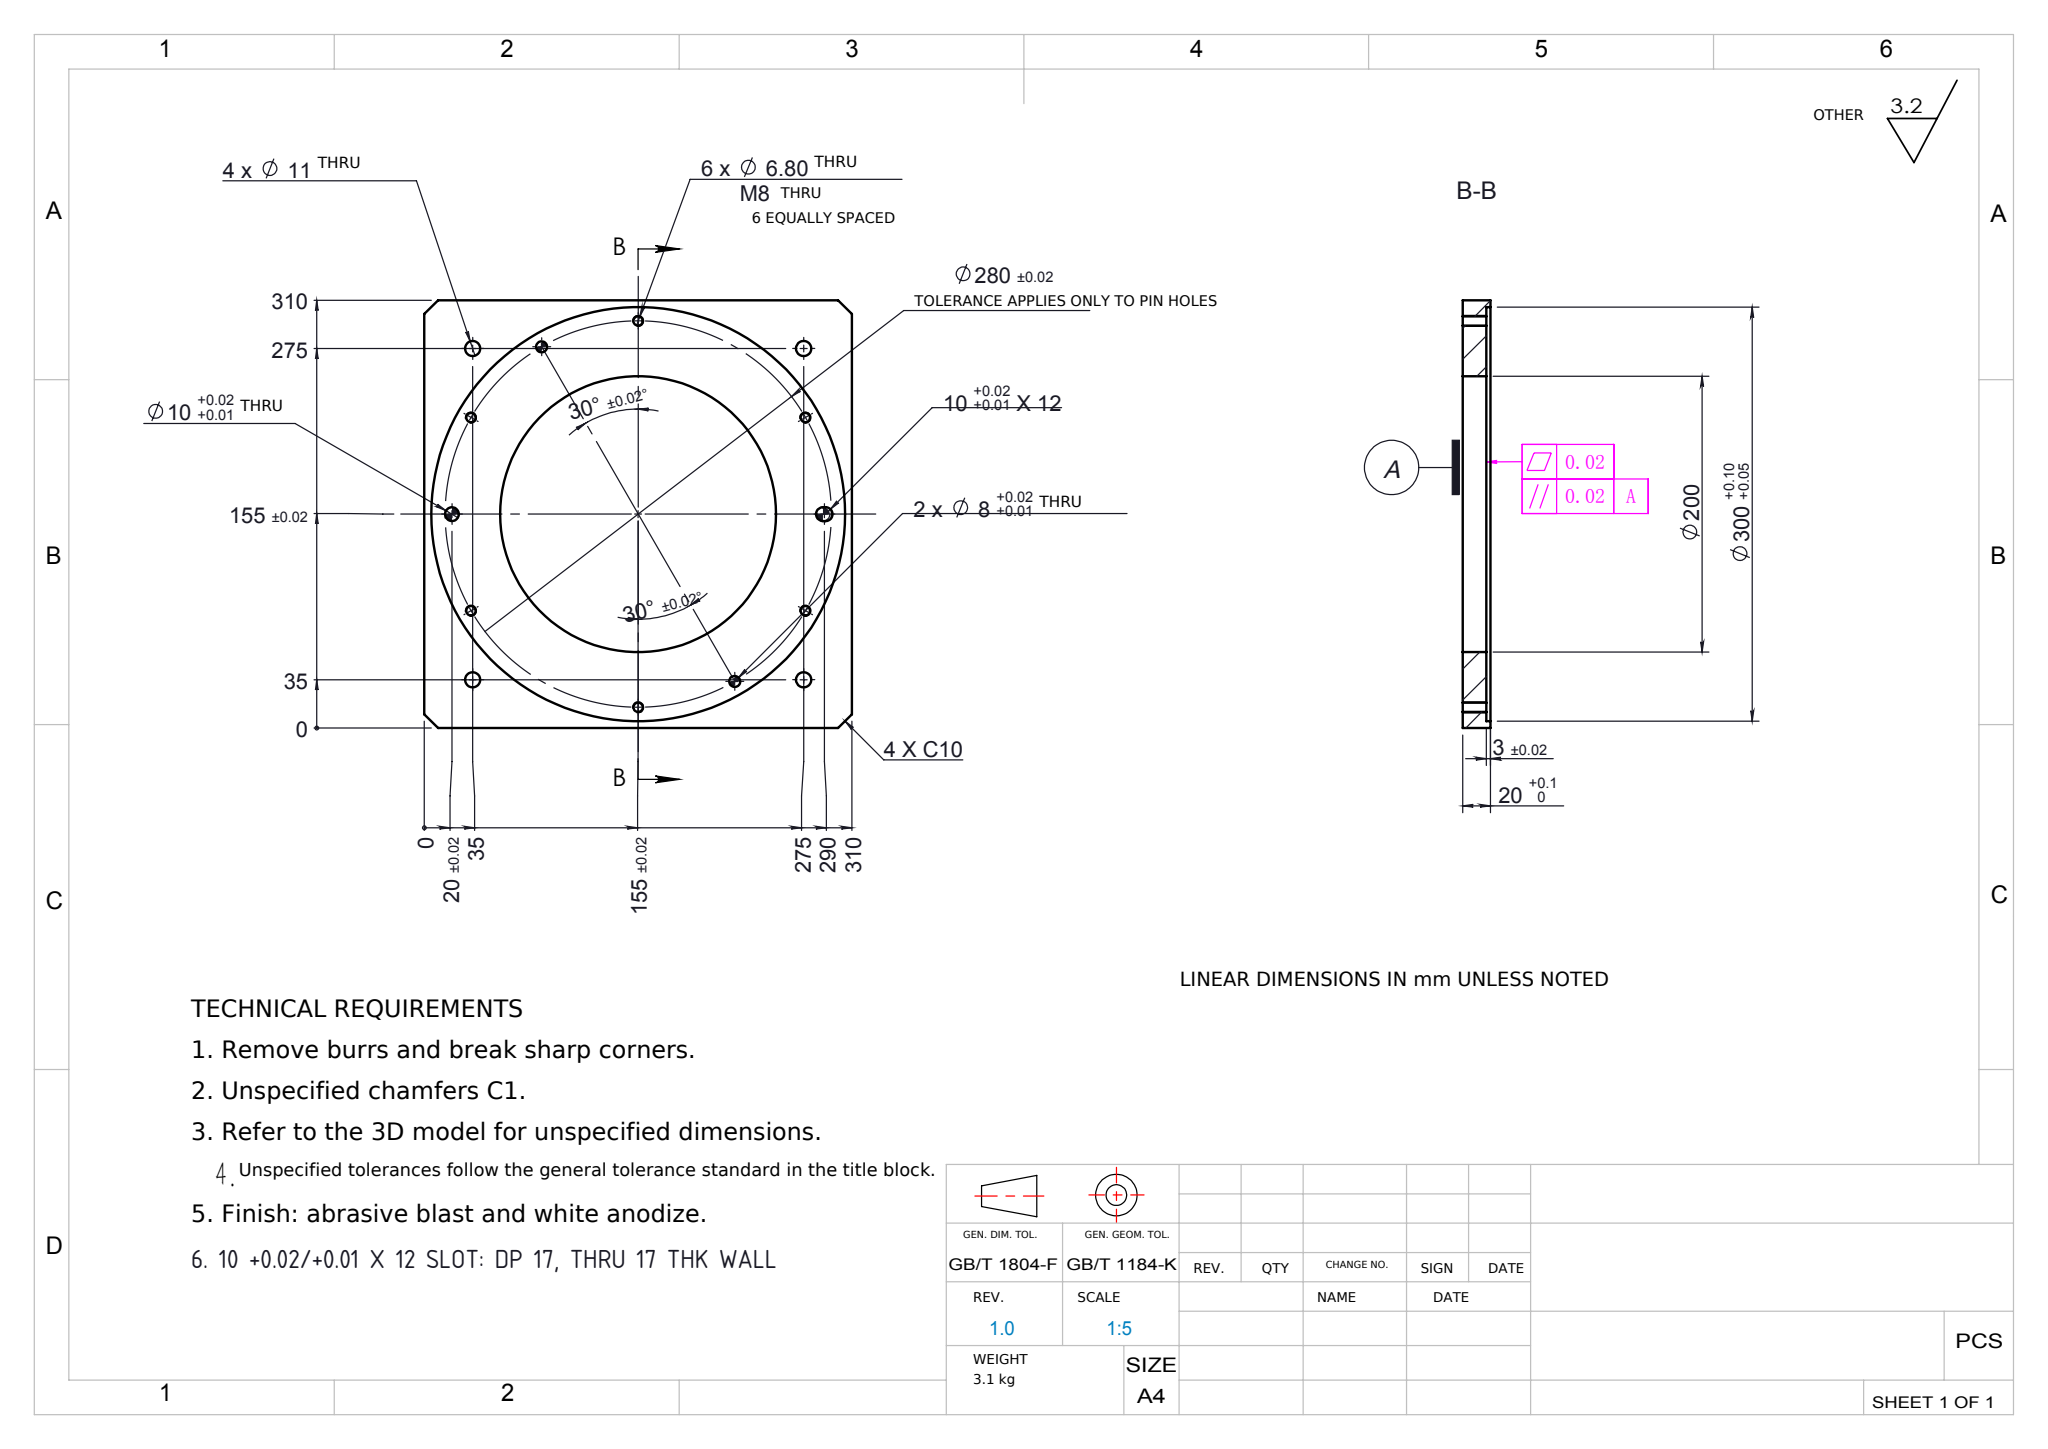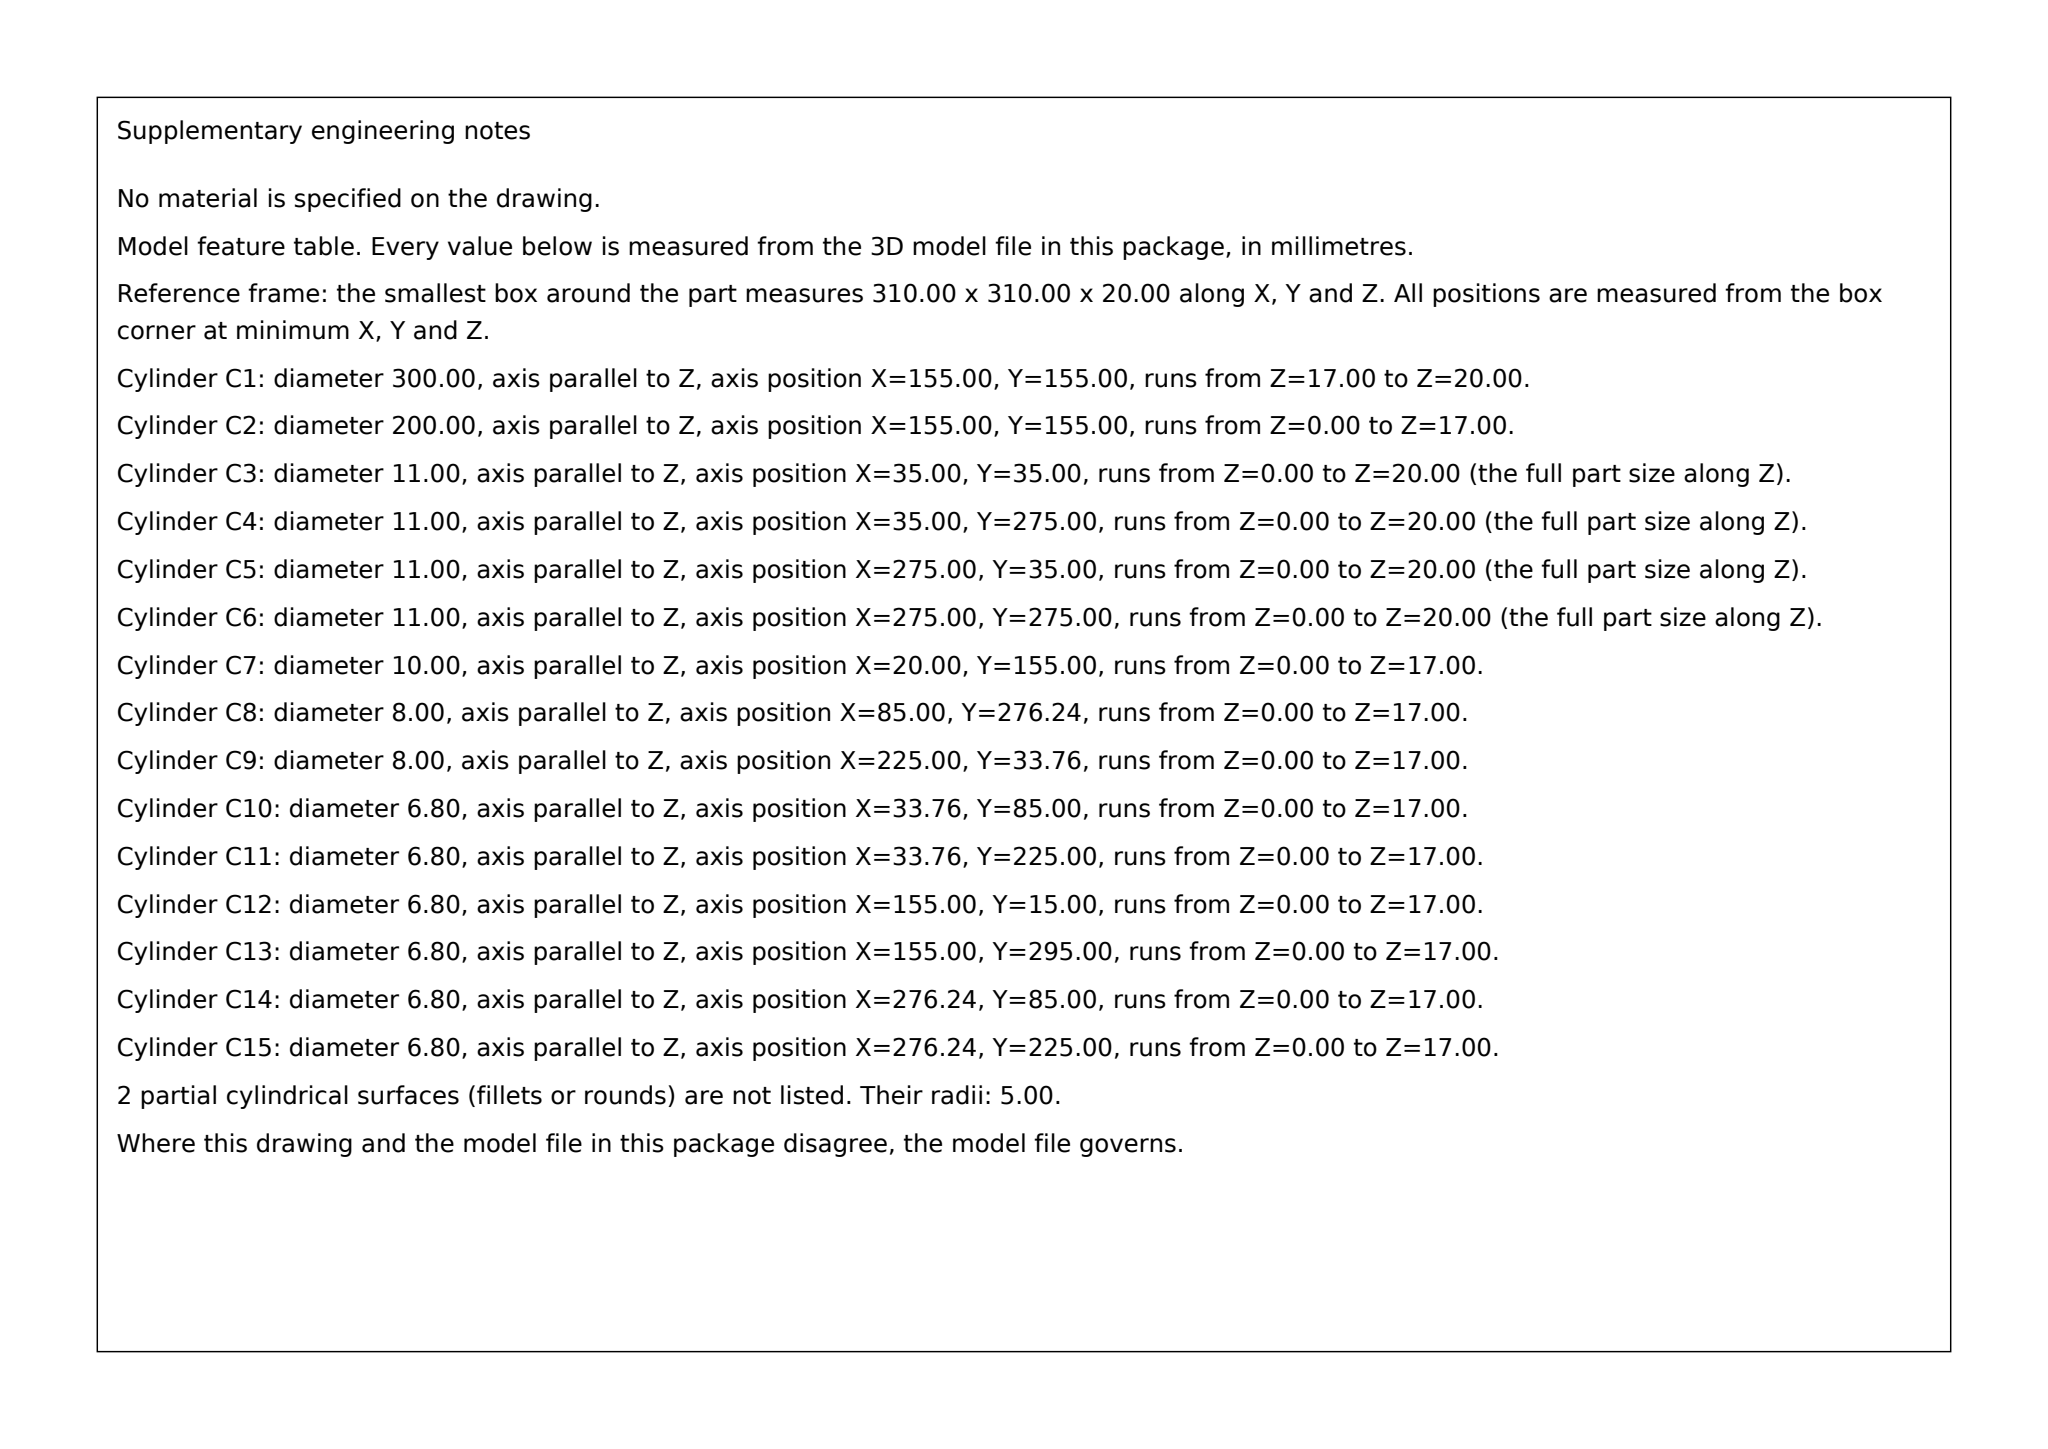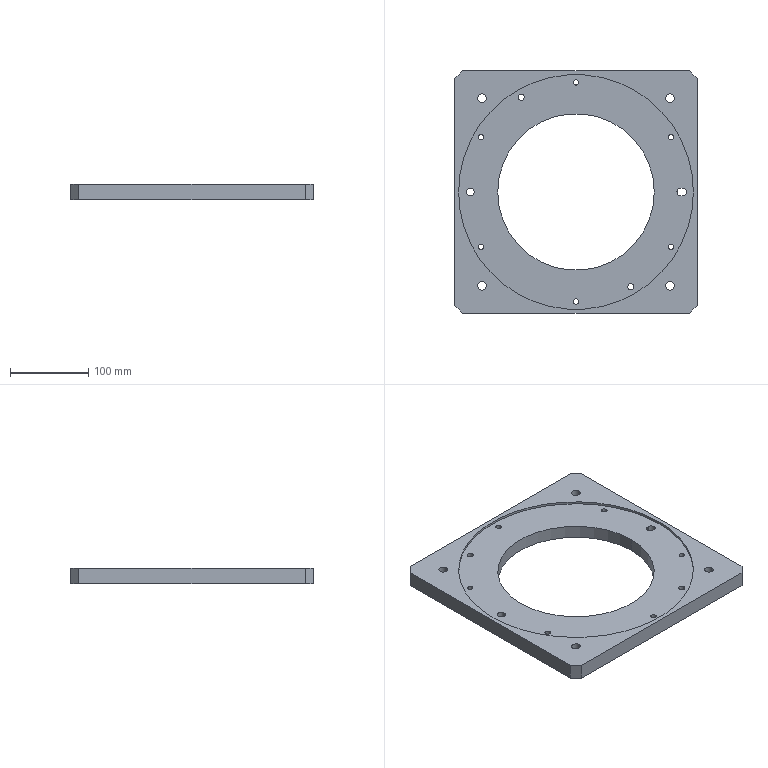Part | SolidWorks | mm | 1 solid | 46 faces | box 310 x 310 x 20 mm | volume 1155845 mm3 | cylinder 33 | plane 13 | commonest cylinder face diameters 6.8 x12 11 x8 10 x5 8 x4 200 x2 300 x2
Drawing notes:
10 +0.02/+0.01 X 12 SLOT: DP 17, THRU 17 THK WALL | from the solid: Ø10 cyls at [289,155] & [291,155], len 17; y-planes 150 & 160 (10 wide); z-planes 0/17/20 give 17 thk wall under 3 thk flange
build123d program:
from build123d import *

# Parameters (mm, degrees)
SKETCH1_W                 = 310
SKETCH1_H                 = 310
BOSS_EXTRUDE1_DEPTH       = 20
SKETCH2_R                 = 150
CUT_EXTRUDE1_DEPTH        = 3
SKETCH3_R                 = 100
CUT_EXTRUDE2_DEPTH        = 220.861
M10_CLEARANCE_HOLE1_D     = 11
CIRPATTERN2_COUNT         = 4
SKETCH11_R                = 5
CUT_EXTRUDE4_DEPTH        = 221.114
CHAMFER1_SIZE             = 10
M8_TAPPED_HOLE1_D         = 6.8
CIRPATTERN3_COUNT         = 6
SIZE_MM_DOWEL_PIN_HOLE2_D = 8


with BuildPart() as part:
    # Sketch1 → Boss-Extrude1 (new body)
    with BuildSketch(Plane.XY):
        Rectangle(SKETCH1_W, SKETCH1_H)
    extrude(amount=BOSS_EXTRUDE1_DEPTH)

    # Sketch2 → Cut-Extrude1 (cut)
    with BuildSketch(Plane.XY.offset(20)):
        Circle(SKETCH2_R)
    extrude(amount=-CUT_EXTRUDE1_DEPTH, mode=Mode.SUBTRACT)

    # Sketch3 → Cut-Extrude2 (cut, through all)
    with BuildSketch(Plane.XY.offset(17)):
        Circle(SKETCH3_R)
    extrude(amount=-CUT_EXTRUDE2_DEPTH, mode=Mode.SUBTRACT)

    # M10 Clearance Hole1 (through all)
    with Locations(Plane(origin=(0, 0, 0), x_dir=(-1, 0, 0), z_dir=(0, 0, -1))):
        with Locations((-120, 120)):
            m10_clearance_hole1 = Hole(M10_CLEARANCE_HOLE1_D / 2)

    # CirPattern2: M10 Clearance Hole1 ×4 about axis
    cirpattern2_axis = Axis((0, 0, 0), (0, 0, 1))
    for i in range(1, CIRPATTERN2_COUNT):
        add(m10_clearance_hole1.rotate(cirpattern2_axis, i * 360 / CIRPATTERN2_COUNT), mode=Mode.SUBTRACT)

    # Sketch11 → Cut-Extrude4 (cut, through all)
    with BuildSketch(Plane(origin=(0, 0, 0), x_dir=(-1, 0, 0), z_dir=(0, 0, -1))):
        with Locations((135, 0)):
            Circle(SKETCH11_R)
        with BuildLine():
            Line((-134, -5), (-136, -5))
            ThreePointArc((-136, -5), (-141, 0), (-136, 5))
            Line((-136, 5), (-134, 5))
            ThreePointArc((-134, 5), (-129, 0), (-134, -5))
        make_face()
    extrude(amount=-CUT_EXTRUDE4_DEPTH, mode=Mode.SUBTRACT)

    # Chamfer1
    chamfer1_edges = [part.edges().sort_by_distance(p)[0] for p in [
        (155, -155, 10),
        (-155, -155, 10),
        (-155, 155, 10),
        (155, 155, 10),
    ]]
    chamfer(chamfer1_edges, length=CHAMFER1_SIZE)

    # M8 Tapped Hole1 (through all)
    with Locations(Plane.XY.offset(17)):
        with Locations((0, 140)):
            m8_tapped_hole1 = Hole(M8_TAPPED_HOLE1_D / 2)

    # CirPattern3: M8 Tapped Hole1 ×6 about axis
    cirpattern3_axis = Axis((0, 0, 0), (0, 0, 1))
    for i in range(1, CIRPATTERN3_COUNT):
        add(m8_tapped_hole1.rotate(cirpattern3_axis, i * 360 / CIRPATTERN3_COUNT), mode=Mode.SUBTRACT)

    # Size mm Dowel Pin Hole2 (through all)
    with Locations(Plane.XY.offset(17)):
        with Locations((-70, 121.244), (70, -121.244)):
            Hole(SIZE_MM_DOWEL_PIN_HOLE2_D / 2)


solid = part.part